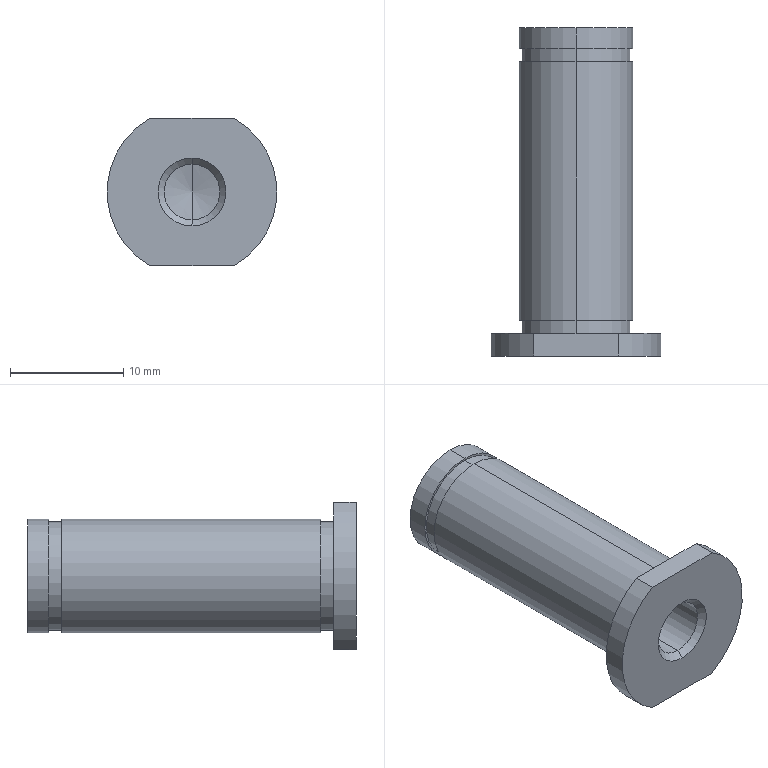Component | SolidWorks | MED02-10-Y2-F24.stp-1 | 1 solid | 24 faces | box 15 x 29 x 13 mm | volume 2240 mm3 | cylinder 12 | plane 8 | cone 4 | commonest cylinder face diameters 9.6 x4 10 x4 4.917 x2 15 x2 | material 45
STEP:
#1=COLOUR_RGB('',0.7922,0.8196,0.9333);
#2=FILL_AREA_STYLE_COLOUR('',#1);
#3=FILL_AREA_STYLE('',(#2));
#4=SURFACE_STYLE_FILL_AREA(#3);
#5=SURFACE_SIDE_STYLE('',(#4));
#6=SURFACE_STYLE_USAGE(.BOTH.,#5);
#7=PRESENTATION_STYLE_ASSIGNMENT((#6));
#8=CARTESIAN_POINT('',(0.5001,-0.1089,18.325));
#9=VERTEX_POINT('',#8);
#10=CARTESIAN_POINT('',(0.5001,-0.1089,18.703));
#11=VERTEX_POINT('',#10);
#12=CARTESIAN_POINT('',(0.5001,-0.1089,18.514));
#13=DIRECTION('',(0.,1.,0.));
#14=DIRECTION('',(0.,-0.,1.));
#15=AXIS2_PLACEMENT_3D('',#12,#13,#14);
#16=CIRCLE('',#15,0.189);
#17=EDGE_CURVE('',#9,#11,#16,.T.);
#18=ORIENTED_EDGE('',*,*,#17,.F.);
#19=CARTESIAN_POINT('',(0.5001,-0.1542,18.325));
#20=VERTEX_POINT('',#19);
#21=CARTESIAN_POINT('',(0.5001,-0.03607,18.325));
#22=DIRECTION('',(-0.,-1.,-0.));
#23=VECTOR('',#22,39.37);
#24=LINE('',#21,#23);
#25=EDGE_CURVE('',#9,#20,#24,.T.);
#26=ORIENTED_EDGE('',*,*,#25,.T.);
#27=CARTESIAN_POINT('',(0.5001,-0.1542,18.703));
#28=VERTEX_POINT('',#27);
#29=CARTESIAN_POINT('',(0.5001,-0.1542,18.514));
#30=DIRECTION('',(0.,1.,0.));
#31=DIRECTION('',(0.,-0.,1.));
#32=AXIS2_PLACEMENT_3D('',#29,#30,#31);
#33=CIRCLE('',#32,0.189);
#34=EDGE_CURVE('',#20,#28,#33,.T.);
#35=ORIENTED_EDGE('',*,*,#34,.T.);
#36=CARTESIAN_POINT('',(0.5001,-0.03607,18.703));
#37=DIRECTION('',(-0.,-1.,-0.));
#38=VECTOR('',#37,39.37);
#39=LINE('',#36,#38);
#40=EDGE_CURVE('',#11,#28,#39,.T.);
#41=ORIENTED_EDGE('',*,*,#40,.F.);
#42=EDGE_LOOP('',(#18,#26,#35,#41));
#43=FACE_OUTER_BOUND('',#42,.T.);
#44=CARTESIAN_POINT('',(0.5001,-0.03607,18.514));
#45=DIRECTION('',(-0.,-1.,-0.));
#46=DIRECTION('',(0.,-0.,1.));
#47=AXIS2_PLACEMENT_3D('',#44,#45,#46);
#48=CYLINDRICAL_SURFACE('',#47,0.189);
#49=ADVANCED_FACE('',(#43),#48,.T.);
#50=CARTESIAN_POINT('',(0.5001,-0.1542,18.317));
#51=VERTEX_POINT('',#50);
#52=CARTESIAN_POINT('',(0.5001,-0.1542,18.711));
#53=VERTEX_POINT('',#52);
#54=CARTESIAN_POINT('',(0.5001,-0.1542,18.514));
#55=DIRECTION('',(0.,1.,0.));
#56=DIRECTION('',(0.,-0.,1.));
#57=AXIS2_PLACEMENT_3D('',#54,#55,#56);
#58=CIRCLE('',#57,0.1969);
#59=EDGE_CURVE('',#51,#53,#58,.T.);
#60=ORIENTED_EDGE('',*,*,#59,.F.);
#61=CARTESIAN_POINT('',(0.5001,-1.054,18.317));
#62=VERTEX_POINT('',#61);
#63=CARTESIAN_POINT('',(0.5001,-0.03607,18.317));
#64=DIRECTION('',(-0.,-1.,-0.));
#65=VECTOR('',#64,39.37);
#66=LINE('',#63,#65);
#67=EDGE_CURVE('',#51,#62,#66,.T.);
#68=ORIENTED_EDGE('',*,*,#67,.T.);
#69=CARTESIAN_POINT('',(0.5001,-1.054,18.711));
#70=VERTEX_POINT('',#69);
#71=CARTESIAN_POINT('',(0.5001,-1.054,18.514));
#72=DIRECTION('',(0.,1.,0.));
#73=DIRECTION('',(0.,-0.,1.));
#74=AXIS2_PLACEMENT_3D('',#71,#72,#73);
#75=CIRCLE('',#74,0.1969);
#76=EDGE_CURVE('',#62,#70,#75,.T.);
#77=ORIENTED_EDGE('',*,*,#76,.T.);
#78=CARTESIAN_POINT('',(0.5001,-0.03607,18.711));
#79=DIRECTION('',(-0.,-1.,-0.));
#80=VECTOR('',#79,39.37);
#81=LINE('',#78,#80);
#82=EDGE_CURVE('',#53,#70,#81,.T.);
#83=ORIENTED_EDGE('',*,*,#82,.F.);
#84=EDGE_LOOP('',(#60,#68,#77,#83));
#85=FACE_OUTER_BOUND('',#84,.T.);
#86=CARTESIAN_POINT('',(0.5001,-0.03607,18.514));
#87=DIRECTION('',(-0.,-1.,-0.));
#88=DIRECTION('',(0.,-0.,1.));
#89=AXIS2_PLACEMENT_3D('',#86,#87,#88);
#90=CYLINDRICAL_SURFACE('',#89,0.1969);
#91=ADVANCED_FACE('',(#85),#90,.T.);
#92=CARTESIAN_POINT('',(0.5001,-1.156,18.417));
#93=VERTEX_POINT('',#92);
#94=CARTESIAN_POINT('',(0.5001,-1.156,18.61));
#95=VERTEX_POINT('',#94);
#96=CARTESIAN_POINT('',(0.5001,-1.156,18.514));
#97=DIRECTION('',(0.,1.,0.));
#98=DIRECTION('',(0.,0.,1.));
#99=AXIS2_PLACEMENT_3D('',#96,#97,#98);
#100=CIRCLE('',#99,0.09679);
#101=EDGE_CURVE('',#93,#95,#100,.T.);
#102=ORIENTED_EDGE('',*,*,#101,.T.);
#103=CARTESIAN_POINT('',(0.5001,-1.178,18.632));
#104=VERTEX_POINT('',#103);
#105=CARTESIAN_POINT('',(0.5001,-1.156,18.61));
#106=DIRECTION('',(0.,-0.7071,0.7071));
#107=VECTOR('',#106,39.37);
#108=LINE('',#105,#107);
#109=EDGE_CURVE('',#95,#104,#108,.T.);
#110=ORIENTED_EDGE('',*,*,#109,.T.);
#111=CARTESIAN_POINT('',(0.5001,-1.178,18.396));
#112=VERTEX_POINT('',#111);
#113=CARTESIAN_POINT('',(0.5001,-1.178,18.514));
#114=DIRECTION('',(0.,1.,0.));
#115=DIRECTION('',(0.,0.,1.));
#116=AXIS2_PLACEMENT_3D('',#113,#114,#115);
#117=CIRCLE('',#116,0.1181);
#118=EDGE_CURVE('',#112,#104,#117,.T.);
#119=ORIENTED_EDGE('',*,*,#118,.F.);
#120=CARTESIAN_POINT('',(0.5001,-1.156,18.417));
#121=DIRECTION('',(-0.,-0.7071,-0.7071));
#122=VECTOR('',#121,39.37);
#123=LINE('',#120,#122);
#124=EDGE_CURVE('',#93,#112,#123,.T.);
#125=ORIENTED_EDGE('',*,*,#124,.F.);
#126=EDGE_LOOP('',(#102,#110,#119,#125));
#127=FACE_OUTER_BOUND('',#126,.T.);
#128=CARTESIAN_POINT('',(0.5001,-1.156,18.514));
#129=DIRECTION('',(-0.,-1.,-0.));
#130=DIRECTION('',(-0.,0.,-1.));
#131=AXIS2_PLACEMENT_3D('',#128,#129,#130);
#132=CONICAL_SURFACE('',#131,0.09679,0.7854);
#133=ADVANCED_FACE('',(#127),#132,.F.);
#134=CARTESIAN_POINT('',(0.5001,-1.054,18.325));
#135=VERTEX_POINT('',#134);
#136=CARTESIAN_POINT('',(0.5001,-1.054,18.703));
#137=VERTEX_POINT('',#136);
#138=CARTESIAN_POINT('',(0.5001,-1.054,18.514));
#139=DIRECTION('',(0.,1.,0.));
#140=DIRECTION('',(0.,-0.,1.));
#141=AXIS2_PLACEMENT_3D('',#138,#139,#140);
#142=CIRCLE('',#141,0.189);
#143=EDGE_CURVE('',#135,#137,#142,.T.);
#144=ORIENTED_EDGE('',*,*,#143,.F.);
#145=CARTESIAN_POINT('',(0.5001,-1.099,18.325));
#146=VERTEX_POINT('',#145);
#147=CARTESIAN_POINT('',(0.5001,-0.03607,18.325));
#148=DIRECTION('',(-0.,-1.,-0.));
#149=VECTOR('',#148,39.37);
#150=LINE('',#147,#149);
#151=EDGE_CURVE('',#135,#146,#150,.T.);
#152=ORIENTED_EDGE('',*,*,#151,.T.);
#153=CARTESIAN_POINT('',(0.5001,-1.099,18.703));
#154=VERTEX_POINT('',#153);
#155=CARTESIAN_POINT('',(0.5001,-1.099,18.514));
#156=DIRECTION('',(0.,1.,0.));
#157=DIRECTION('',(0.,-0.,1.));
#158=AXIS2_PLACEMENT_3D('',#155,#156,#157);
#159=CIRCLE('',#158,0.189);
#160=EDGE_CURVE('',#146,#154,#159,.T.);
#161=ORIENTED_EDGE('',*,*,#160,.T.);
#162=CARTESIAN_POINT('',(0.5001,-0.03607,18.703));
#163=DIRECTION('',(-0.,-1.,-0.));
#164=VECTOR('',#163,39.37);
#165=LINE('',#162,#164);
#166=EDGE_CURVE('',#137,#154,#165,.T.);
#167=ORIENTED_EDGE('',*,*,#166,.F.);
#168=EDGE_LOOP('',(#144,#152,#161,#167));
#169=FACE_OUTER_BOUND('',#168,.T.);
#170=CARTESIAN_POINT('',(0.5001,-0.03607,18.514));
#171=DIRECTION('',(-0.,-1.,-0.));
#172=DIRECTION('',(0.,-0.,1.));
#173=AXIS2_PLACEMENT_3D('',#170,#171,#172);
#174=CYLINDRICAL_SURFACE('',#173,0.189);
#175=ADVANCED_FACE('',(#169),#174,.T.);
#176=CARTESIAN_POINT('',(0.5001,-0.7762,18.61));
#177=VERTEX_POINT('',#176);
#178=CARTESIAN_POINT('',(0.5001,-0.7762,18.417));
#179=VERTEX_POINT('',#178);
#180=CARTESIAN_POINT('',(0.5001,-0.7762,18.514));
#181=DIRECTION('',(0.,1.,0.));
#182=DIRECTION('',(0.,0.,1.));
#183=AXIS2_PLACEMENT_3D('',#180,#181,#182);
#184=CIRCLE('',#183,0.09679);
#185=EDGE_CURVE('',#177,#179,#184,.T.);
#186=ORIENTED_EDGE('',*,*,#185,.T.);
#187=CARTESIAN_POINT('',(0.5001,-0.03607,18.417));
#188=DIRECTION('',(-0.,-1.,-0.));
#189=VECTOR('',#188,39.37);
#190=LINE('',#187,#189);
#191=EDGE_CURVE('',#179,#93,#190,.T.);
#192=ORIENTED_EDGE('',*,*,#191,.T.);
#193=CARTESIAN_POINT('',(0.5001,-1.156,18.514));
#194=DIRECTION('',(0.,1.,0.));
#195=DIRECTION('',(0.,0.,1.));
#196=AXIS2_PLACEMENT_3D('',#193,#194,#195);
#197=CIRCLE('',#196,0.09679);
#198=EDGE_CURVE('',#95,#93,#197,.T.);
#199=ORIENTED_EDGE('',*,*,#198,.F.);
#200=CARTESIAN_POINT('',(0.5001,-0.03607,18.61));
#201=DIRECTION('',(-0.,-1.,-0.));
#202=VECTOR('',#201,39.37);
#203=LINE('',#200,#202);
#204=EDGE_CURVE('',#177,#95,#203,.T.);
#205=ORIENTED_EDGE('',*,*,#204,.F.);
#206=EDGE_LOOP('',(#186,#192,#199,#205));
#207=FACE_OUTER_BOUND('',#206,.T.);
#208=CARTESIAN_POINT('',(0.5001,-0.03607,18.514));
#209=DIRECTION('',(-0.,-1.,-0.));
#210=DIRECTION('',(0.,-0.,1.));
#211=AXIS2_PLACEMENT_3D('',#208,#209,#210);
#212=CYLINDRICAL_SURFACE('',#211,0.09679);
#213=ADVANCED_FACE('',(#207),#212,.F.);
#214=CARTESIAN_POINT('',(0.5001,-0.03607,18.317));
#215=VERTEX_POINT('',#214);
#216=CARTESIAN_POINT('',(0.5001,-0.03607,18.711));
#217=VERTEX_POINT('',#216);
#218=CARTESIAN_POINT('',(0.5001,-0.03607,18.514));
#219=DIRECTION('',(0.,1.,0.));
#220=DIRECTION('',(0.,-0.,1.));
#221=AXIS2_PLACEMENT_3D('',#218,#219,#220);
#222=CIRCLE('',#221,0.1969);
#223=EDGE_CURVE('',#215,#217,#222,.T.);
#224=ORIENTED_EDGE('',*,*,#223,.F.);
#225=CARTESIAN_POINT('',(0.5001,-0.1089,18.317));
#226=VERTEX_POINT('',#225);
#227=CARTESIAN_POINT('',(0.5001,-0.03607,18.317));
#228=DIRECTION('',(-0.,-1.,-0.));
#229=VECTOR('',#228,39.37);
#230=LINE('',#227,#229);
#231=EDGE_CURVE('',#215,#226,#230,.T.);
#232=ORIENTED_EDGE('',*,*,#231,.T.);
#233=CARTESIAN_POINT('',(0.5001,-0.1089,18.711));
#234=VERTEX_POINT('',#233);
#235=CARTESIAN_POINT('',(0.5001,-0.1089,18.514));
#236=DIRECTION('',(0.,1.,0.));
#237=DIRECTION('',(0.,-0.,1.));
#238=AXIS2_PLACEMENT_3D('',#235,#236,#237);
#239=CIRCLE('',#238,0.1969);
#240=EDGE_CURVE('',#226,#234,#239,.T.);
#241=ORIENTED_EDGE('',*,*,#240,.T.);
#242=CARTESIAN_POINT('',(0.5001,-0.03607,18.711));
#243=DIRECTION('',(-0.,-1.,-0.));
#244=VECTOR('',#243,39.37);
#245=LINE('',#242,#244);
#246=EDGE_CURVE('',#217,#234,#245,.T.);
#247=ORIENTED_EDGE('',*,*,#246,.F.);
#248=EDGE_LOOP('',(#224,#232,#241,#247));
#249=FACE_OUTER_BOUND('',#248,.T.);
#250=CARTESIAN_POINT('',(0.5001,-0.03607,18.514));
#251=DIRECTION('',(-0.,-1.,-0.));
#252=DIRECTION('',(0.,-0.,1.));
#253=AXIS2_PLACEMENT_3D('',#250,#251,#252);
#254=CYLINDRICAL_SURFACE('',#253,0.1969);
#255=ADVANCED_FACE('',(#249),#254,.T.);
#256=CARTESIAN_POINT('',(0.5001,-0.7565,18.514));
#257=VERTEX_POINT('',#256);
#258=CARTESIAN_POINT('',(0.5001,-8.603,-20.067));
#259=DIRECTION('',(-0.,-0.1993,-0.9799));
#260=VECTOR('',#259,39.37);
#261=LINE('',#258,#260);
#262=EDGE_CURVE('',#257,#179,#261,.T.);
#263=ORIENTED_EDGE('',*,*,#262,.F.);
#264=CARTESIAN_POINT('',(0.5001,-8.603,57.094));
#265=DIRECTION('',(0.,-0.1993,0.9799));
#266=VECTOR('',#265,39.37);
#267=LINE('',#264,#266);
#268=EDGE_CURVE('',#257,#177,#267,.T.);
#269=ORIENTED_EDGE('',*,*,#268,.T.);
#270=CARTESIAN_POINT('',(0.5001,-0.7762,18.514));
#271=DIRECTION('',(0.,1.,0.));
#272=DIRECTION('',(0.,0.,1.));
#273=AXIS2_PLACEMENT_3D('',#270,#271,#272);
#274=CIRCLE('',#273,0.09679);
#275=EDGE_CURVE('',#179,#177,#274,.T.);
#276=ORIENTED_EDGE('',*,*,#275,.F.);
#277=EDGE_LOOP('',(#263,#269,#276));
#278=FACE_OUTER_BOUND('',#277,.T.);
#279=CARTESIAN_POINT('',(0.5001,-8.603,18.514));
#280=DIRECTION('',(-0.,-1.,-0.));
#281=DIRECTION('',(-0.,0.,-1.));
#282=AXIS2_PLACEMENT_3D('',#279,#280,#281);
#283=CONICAL_SURFACE('',#282,38.58,1.37);
#284=ADVANCED_FACE('',(#278),#283,.F.);
#285=CARTESIAN_POINT('',(0.3528,-1.178,18.258));
#286=VERTEX_POINT('',#285);
#287=CARTESIAN_POINT('',(0.3528,-1.178,18.77));
#288=VERTEX_POINT('',#287);
#289=CARTESIAN_POINT('',(0.5001,-1.178,18.514));
#290=DIRECTION('',(0.,1.,0.));
#291=DIRECTION('',(0.,-0.,1.));
#292=AXIS2_PLACEMENT_3D('',#289,#290,#291);
#293=CIRCLE('',#292,0.2953);
#294=EDGE_CURVE('',#286,#288,#293,.T.);
#295=ORIENTED_EDGE('',*,*,#294,.T.);
#296=CARTESIAN_POINT('',(0.3528,-1.099,18.77));
#297=VERTEX_POINT('',#296);
#298=CARTESIAN_POINT('',(0.3528,-0.03607,18.77));
#299=DIRECTION('',(0.,1.,0.));
#300=VECTOR('',#299,39.37);
#301=LINE('',#298,#300);
#302=EDGE_CURVE('',#288,#297,#301,.T.);
#303=ORIENTED_EDGE('',*,*,#302,.T.);
#304=CARTESIAN_POINT('',(0.3528,-1.099,18.258));
#305=VERTEX_POINT('',#304);
#306=CARTESIAN_POINT('',(0.5001,-1.099,18.514));
#307=DIRECTION('',(0.,1.,0.));
#308=DIRECTION('',(0.,-0.,1.));
#309=AXIS2_PLACEMENT_3D('',#306,#307,#308);
#310=CIRCLE('',#309,0.2953);
#311=EDGE_CURVE('',#305,#297,#310,.T.);
#312=ORIENTED_EDGE('',*,*,#311,.F.);
#313=CARTESIAN_POINT('',(0.3528,-0.03607,18.258));
#314=DIRECTION('',(-0.,-1.,-0.));
#315=VECTOR('',#314,39.37);
#316=LINE('',#313,#315);
#317=EDGE_CURVE('',#305,#286,#316,.T.);
#318=ORIENTED_EDGE('',*,*,#317,.T.);
#319=EDGE_LOOP('',(#295,#303,#312,#318));
#320=FACE_OUTER_BOUND('',#319,.T.);
#321=CARTESIAN_POINT('',(0.5001,-0.03607,18.514));
#322=DIRECTION('',(-0.,-1.,-0.));
#323=DIRECTION('',(0.,-0.,1.));
#324=AXIS2_PLACEMENT_3D('',#321,#322,#323);
#325=CYLINDRICAL_SURFACE('',#324,0.2953);
#326=ADVANCED_FACE('',(#320),#325,.T.);
#327=ORIENTED_EDGE('',*,*,#268,.F.);
#328=ORIENTED_EDGE('',*,*,#262,.T.);
#329=ORIENTED_EDGE('',*,*,#185,.F.);
#330=EDGE_LOOP('',(#327,#328,#329));
#331=FACE_OUTER_BOUND('',#330,.T.);
#332=CARTESIAN_POINT('',(0.5001,-8.603,18.514));
#333=DIRECTION('',(-0.,-1.,-0.));
#334=DIRECTION('',(-0.,0.,-1.));
#335=AXIS2_PLACEMENT_3D('',#332,#333,#334);
#336=CONICAL_SURFACE('',#335,38.58,1.37);
#337=ADVANCED_FACE('',(#331),#336,.F.);
#338=CARTESIAN_POINT('',(0.6474,-1.178,18.77));
#339=VERTEX_POINT('',#338);
#340=CARTESIAN_POINT('',(0.2049,-1.178,18.77));
#341=DIRECTION('',(1.,-0.,-0.));
#342=VECTOR('',#341,39.37);
#343=LINE('',#340,#342);
#344=EDGE_CURVE('',#288,#339,#343,.T.);
#345=ORIENTED_EDGE('',*,*,#344,.T.);
#346=CARTESIAN_POINT('',(0.6474,-1.099,18.77));
#347=VERTEX_POINT('',#346);
#348=CARTESIAN_POINT('',(0.6474,-0.03607,18.77));
#349=DIRECTION('',(-0.,-1.,-0.));
#350=VECTOR('',#349,39.37);
#351=LINE('',#348,#350);
#352=EDGE_CURVE('',#347,#339,#351,.T.);
#353=ORIENTED_EDGE('',*,*,#352,.F.);
#354=CARTESIAN_POINT('',(0.7954,-1.099,18.77));
#355=DIRECTION('',(1.,-0.,-0.));
#356=VECTOR('',#355,39.37);
#357=LINE('',#354,#356);
#358=EDGE_CURVE('',#297,#347,#357,.T.);
#359=ORIENTED_EDGE('',*,*,#358,.F.);
#360=ORIENTED_EDGE('',*,*,#302,.F.);
#361=EDGE_LOOP('',(#345,#353,#359,#360));
#362=FACE_OUTER_BOUND('',#361,.T.);
#363=CARTESIAN_POINT('',(0.2049,-1.099,18.77));
#364=DIRECTION('',(-0.,0.,-1.));
#365=DIRECTION('',(1.,-0.,-0.));
#366=AXIS2_PLACEMENT_3D('',#363,#364,#365);
#367=PLANE('',#366);
#368=ADVANCED_FACE('',(#362),#367,.F.);
#369=CARTESIAN_POINT('',(0.6474,-1.178,18.258));
#370=VERTEX_POINT('',#369);
#371=CARTESIAN_POINT('',(0.5001,-1.178,18.514));
#372=DIRECTION('',(0.,1.,0.));
#373=DIRECTION('',(0.,-0.,1.));
#374=AXIS2_PLACEMENT_3D('',#371,#372,#373);
#375=CIRCLE('',#374,0.2953);
#376=EDGE_CURVE('',#339,#370,#375,.T.);
#377=ORIENTED_EDGE('',*,*,#376,.F.);
#378=ORIENTED_EDGE('',*,*,#344,.F.);
#379=ORIENTED_EDGE('',*,*,#294,.F.);
#380=CARTESIAN_POINT('',(0.7954,-1.178,18.258));
#381=DIRECTION('',(-1.,0.,0.));
#382=VECTOR('',#381,39.37);
#383=LINE('',#380,#382);
#384=EDGE_CURVE('',#370,#286,#383,.T.);
#385=ORIENTED_EDGE('',*,*,#384,.F.);
#386=EDGE_LOOP('',(#377,#378,#379,#385));
#387=FACE_OUTER_BOUND('',#386,.T.);
#388=ORIENTED_EDGE('',*,*,#118,.T.);
#389=CARTESIAN_POINT('',(0.5001,-1.178,18.514));
#390=DIRECTION('',(0.,1.,0.));
#391=DIRECTION('',(0.,0.,1.));
#392=AXIS2_PLACEMENT_3D('',#389,#390,#391);
#393=CIRCLE('',#392,0.1181);
#394=EDGE_CURVE('',#104,#112,#393,.T.);
#395=ORIENTED_EDGE('',*,*,#394,.T.);
#396=EDGE_LOOP('',(#388,#395));
#397=FACE_BOUND('',#396,.T.);
#398=CARTESIAN_POINT('',(0.6182,-1.178,18.514));
#399=DIRECTION('',(0.,1.,0.));
#400=DIRECTION('',(-1.,0.,0.));
#401=AXIS2_PLACEMENT_3D('',#398,#399,#400);
#402=PLANE('',#401);
#403=ADVANCED_FACE('',(#387,#397),#402,.F.);
#404=ORIENTED_EDGE('',*,*,#311,.T.);
#405=ORIENTED_EDGE('',*,*,#358,.T.);
#406=CARTESIAN_POINT('',(0.6474,-1.099,18.258));
#407=VERTEX_POINT('',#406);
#408=CARTESIAN_POINT('',(0.5001,-1.099,18.514));
#409=DIRECTION('',(0.,1.,0.));
#410=DIRECTION('',(0.,-0.,1.));
#411=AXIS2_PLACEMENT_3D('',#408,#409,#410);
#412=CIRCLE('',#411,0.2953);
#413=EDGE_CURVE('',#347,#407,#412,.T.);
#414=ORIENTED_EDGE('',*,*,#413,.T.);
#415=CARTESIAN_POINT('',(0.7954,-1.099,18.258));
#416=DIRECTION('',(-1.,0.,0.));
#417=VECTOR('',#416,39.37);
#418=LINE('',#415,#417);
#419=EDGE_CURVE('',#407,#305,#418,.T.);
#420=ORIENTED_EDGE('',*,*,#419,.T.);
#421=EDGE_LOOP('',(#404,#405,#414,#420));
#422=FACE_OUTER_BOUND('',#421,.T.);
#423=CARTESIAN_POINT('',(0.5001,-1.099,18.514));
#424=DIRECTION('',(0.,1.,0.));
#425=DIRECTION('',(0.,-0.,1.));
#426=AXIS2_PLACEMENT_3D('',#423,#424,#425);
#427=CIRCLE('',#426,0.189);
#428=EDGE_CURVE('',#154,#146,#427,.T.);
#429=ORIENTED_EDGE('',*,*,#428,.F.);
#430=ORIENTED_EDGE('',*,*,#160,.F.);
#431=EDGE_LOOP('',(#429,#430));
#432=FACE_BOUND('',#431,.T.);
#433=CARTESIAN_POINT('',(0.7954,-1.099,18.514));
#434=DIRECTION('',(-0.,-1.,-0.));
#435=DIRECTION('',(-0.,0.,-1.));
#436=AXIS2_PLACEMENT_3D('',#433,#434,#435);
#437=PLANE('',#436);
#438=ADVANCED_FACE('',(#422,#432),#437,.F.);
#439=ORIENTED_EDGE('',*,*,#376,.T.);
#440=CARTESIAN_POINT('',(0.6474,-0.03607,18.258));
#441=DIRECTION('',(0.,1.,0.));
#442=VECTOR('',#441,39.37);
#443=LINE('',#440,#442);
#444=EDGE_CURVE('',#370,#407,#443,.T.);
#445=ORIENTED_EDGE('',*,*,#444,.T.);
#446=ORIENTED_EDGE('',*,*,#413,.F.);
#447=ORIENTED_EDGE('',*,*,#352,.T.);
#448=EDGE_LOOP('',(#439,#445,#446,#447));
#449=FACE_OUTER_BOUND('',#448,.T.);
#450=CARTESIAN_POINT('',(0.5001,-0.03607,18.514));
#451=DIRECTION('',(-0.,-1.,-0.));
#452=DIRECTION('',(0.,-0.,1.));
#453=AXIS2_PLACEMENT_3D('',#450,#451,#452);
#454=CYLINDRICAL_SURFACE('',#453,0.2953);
#455=ADVANCED_FACE('',(#449),#454,.T.);
#456=ORIENTED_EDGE('',*,*,#384,.T.);
#457=ORIENTED_EDGE('',*,*,#317,.F.);
#458=ORIENTED_EDGE('',*,*,#419,.F.);
#459=ORIENTED_EDGE('',*,*,#444,.F.);
#460=EDGE_LOOP('',(#456,#457,#458,#459));
#461=FACE_OUTER_BOUND('',#460,.T.);
#462=CARTESIAN_POINT('',(0.7954,-1.099,18.258));
#463=DIRECTION('',(0.,-0.,1.));
#464=DIRECTION('',(-0.,-1.,-0.));
#465=AXIS2_PLACEMENT_3D('',#462,#463,#464);
#466=PLANE('',#465);
#467=ADVANCED_FACE('',(#461),#466,.F.);
#468=CARTESIAN_POINT('',(0.5001,-0.03607,18.514));
#469=DIRECTION('',(0.,1.,0.));
#470=DIRECTION('',(0.,-0.,1.));
#471=AXIS2_PLACEMENT_3D('',#468,#469,#470);
#472=CIRCLE('',#471,0.1969);
#473=EDGE_CURVE('',#217,#215,#472,.T.);
#474=ORIENTED_EDGE('',*,*,#473,.T.);
#475=ORIENTED_EDGE('',*,*,#223,.T.);
#476=EDGE_LOOP('',(#474,#475));
#477=FACE_OUTER_BOUND('',#476,.T.);
#478=CARTESIAN_POINT('',(0.697,-0.03607,18.514));
#479=DIRECTION('',(-0.,-1.,-0.));
#480=DIRECTION('',(-0.,0.,-1.));
#481=AXIS2_PLACEMENT_3D('',#478,#479,#480);
#482=PLANE('',#481);
#483=ADVANCED_FACE('',(#477),#482,.F.);
#484=ORIENTED_EDGE('',*,*,#231,.F.);
#485=ORIENTED_EDGE('',*,*,#473,.F.);
#486=ORIENTED_EDGE('',*,*,#246,.T.);
#487=CARTESIAN_POINT('',(0.5001,-0.1089,18.514));
#488=DIRECTION('',(0.,1.,0.));
#489=DIRECTION('',(0.,-0.,1.));
#490=AXIS2_PLACEMENT_3D('',#487,#488,#489);
#491=CIRCLE('',#490,0.1969);
#492=EDGE_CURVE('',#234,#226,#491,.T.);
#493=ORIENTED_EDGE('',*,*,#492,.T.);
#494=EDGE_LOOP('',(#484,#485,#486,#493));
#495=FACE_OUTER_BOUND('',#494,.T.);
#496=CARTESIAN_POINT('',(0.5001,-0.03607,18.514));
#497=DIRECTION('',(-0.,-1.,-0.));
#498=DIRECTION('',(0.,-0.,1.));
#499=AXIS2_PLACEMENT_3D('',#496,#497,#498);
#500=CYLINDRICAL_SURFACE('',#499,0.1969);
#501=ADVANCED_FACE('',(#495),#500,.T.);
#502=ORIENTED_EDGE('',*,*,#191,.F.);
#503=ORIENTED_EDGE('',*,*,#275,.T.);
#504=ORIENTED_EDGE('',*,*,#204,.T.);
#505=ORIENTED_EDGE('',*,*,#101,.F.);
#506=EDGE_LOOP('',(#502,#503,#504,#505));
#507=FACE_OUTER_BOUND('',#506,.T.);
#508=CARTESIAN_POINT('',(0.5001,-0.03607,18.514));
#509=DIRECTION('',(-0.,-1.,-0.));
#510=DIRECTION('',(0.,-0.,1.));
#511=AXIS2_PLACEMENT_3D('',#508,#509,#510);
#512=CYLINDRICAL_SURFACE('',#511,0.09679);
#513=ADVANCED_FACE('',(#507),#512,.F.);
#514=ORIENTED_EDGE('',*,*,#151,.F.);
#515=CARTESIAN_POINT('',(0.5001,-1.054,18.514));
#516=DIRECTION('',(0.,1.,0.));
#517=DIRECTION('',(0.,-0.,1.));
#518=AXIS2_PLACEMENT_3D('',#515,#516,#517);
#519=CIRCLE('',#518,0.189);
#520=EDGE_CURVE('',#137,#135,#519,.T.);
#521=ORIENTED_EDGE('',*,*,#520,.F.);
#522=ORIENTED_EDGE('',*,*,#166,.T.);
#523=ORIENTED_EDGE('',*,*,#428,.T.);
#524=EDGE_LOOP('',(#514,#521,#522,#523));
#525=FACE_OUTER_BOUND('',#524,.T.);
#526=CARTESIAN_POINT('',(0.5001,-0.03607,18.514));
#527=DIRECTION('',(-0.,-1.,-0.));
#528=DIRECTION('',(0.,-0.,1.));
#529=AXIS2_PLACEMENT_3D('',#526,#527,#528);
#530=CYLINDRICAL_SURFACE('',#529,0.189);
#531=ADVANCED_FACE('',(#525),#530,.T.);
#532=ORIENTED_EDGE('',*,*,#109,.F.);
#533=ORIENTED_EDGE('',*,*,#198,.T.);
#534=ORIENTED_EDGE('',*,*,#124,.T.);
#535=ORIENTED_EDGE('',*,*,#394,.F.);
#536=EDGE_LOOP('',(#532,#533,#534,#535));
#537=FACE_OUTER_BOUND('',#536,.T.);
#538=CARTESIAN_POINT('',(0.5001,-1.156,18.514));
#539=DIRECTION('',(-0.,-1.,-0.));
#540=DIRECTION('',(-0.,0.,-1.));
#541=AXIS2_PLACEMENT_3D('',#538,#539,#540);
#542=CONICAL_SURFACE('',#541,0.09679,0.7854);
#543=ADVANCED_FACE('',(#537),#542,.F.);
#544=CARTESIAN_POINT('',(0.5001,-1.054,18.514));
#545=DIRECTION('',(0.,1.,0.));
#546=DIRECTION('',(0.,-0.,1.));
#547=AXIS2_PLACEMENT_3D('',#544,#545,#546);
#548=CIRCLE('',#547,0.1969);
#549=EDGE_CURVE('',#70,#62,#548,.T.);
#550=ORIENTED_EDGE('',*,*,#549,.F.);
#551=ORIENTED_EDGE('',*,*,#76,.F.);
#552=EDGE_LOOP('',(#550,#551));
#553=FACE_OUTER_BOUND('',#552,.T.);
#554=ORIENTED_EDGE('',*,*,#520,.T.);
#555=ORIENTED_EDGE('',*,*,#143,.T.);
#556=EDGE_LOOP('',(#554,#555));
#557=FACE_BOUND('',#556,.T.);
#558=CARTESIAN_POINT('',(0.6891,-1.054,18.514));
#559=DIRECTION('',(0.,1.,0.));
#560=DIRECTION('',(-1.,0.,0.));
#561=AXIS2_PLACEMENT_3D('',#558,#559,#560);
#562=PLANE('',#561);
#563=ADVANCED_FACE('',(#553,#557),#562,.F.);
#564=ORIENTED_EDGE('',*,*,#67,.F.);
#565=CARTESIAN_POINT('',(0.5001,-0.1542,18.514));
#566=DIRECTION('',(0.,1.,0.));
#567=DIRECTION('',(0.,-0.,1.));
#568=AXIS2_PLACEMENT_3D('',#565,#566,#567);
#569=CIRCLE('',#568,0.1969);
#570=EDGE_CURVE('',#53,#51,#569,.T.);
#571=ORIENTED_EDGE('',*,*,#570,.F.);
#572=ORIENTED_EDGE('',*,*,#82,.T.);
#573=ORIENTED_EDGE('',*,*,#549,.T.);
#574=EDGE_LOOP('',(#564,#571,#572,#573));
#575=FACE_OUTER_BOUND('',#574,.T.);
#576=CARTESIAN_POINT('',(0.5001,-0.03607,18.514));
#577=DIRECTION('',(-0.,-1.,-0.));
#578=DIRECTION('',(0.,-0.,1.));
#579=AXIS2_PLACEMENT_3D('',#576,#577,#578);
#580=CYLINDRICAL_SURFACE('',#579,0.1969);
#581=ADVANCED_FACE('',(#575),#580,.T.);
#582=ORIENTED_EDGE('',*,*,#570,.T.);
#583=ORIENTED_EDGE('',*,*,#59,.T.);
#584=EDGE_LOOP('',(#582,#583));
#585=FACE_OUTER_BOUND('',#584,.T.);
#586=CARTESIAN_POINT('',(0.5001,-0.1542,18.514));
#587=DIRECTION('',(0.,1.,0.));
#588=DIRECTION('',(0.,-0.,1.));
#589=AXIS2_PLACEMENT_3D('',#586,#587,#588);
#590=CIRCLE('',#589,0.189);
#591=EDGE_CURVE('',#28,#20,#590,.T.);
#592=ORIENTED_EDGE('',*,*,#591,.F.);
#593=ORIENTED_EDGE('',*,*,#34,.F.);
#594=EDGE_LOOP('',(#592,#593));
#595=FACE_BOUND('',#594,.T.);
#596=CARTESIAN_POINT('',(0.697,-0.1542,18.514));
#597=DIRECTION('',(-0.,-1.,-0.));
#598=DIRECTION('',(-0.,0.,-1.));
#599=AXIS2_PLACEMENT_3D('',#596,#597,#598);
#600=PLANE('',#599);
#601=ADVANCED_FACE('',(#585,#595),#600,.F.);
#602=ORIENTED_EDGE('',*,*,#25,.F.);
#603=CARTESIAN_POINT('',(0.5001,-0.1089,18.514));
#604=DIRECTION('',(0.,1.,0.));
#605=DIRECTION('',(0.,-0.,1.));
#606=AXIS2_PLACEMENT_3D('',#603,#604,#605);
#607=CIRCLE('',#606,0.189);
#608=EDGE_CURVE('',#11,#9,#607,.T.);
#609=ORIENTED_EDGE('',*,*,#608,.F.);
#610=ORIENTED_EDGE('',*,*,#40,.T.);
#611=ORIENTED_EDGE('',*,*,#591,.T.);
#612=EDGE_LOOP('',(#602,#609,#610,#611));
#613=FACE_OUTER_BOUND('',#612,.T.);
#614=CARTESIAN_POINT('',(0.5001,-0.03607,18.514));
#615=DIRECTION('',(-0.,-1.,-0.));
#616=DIRECTION('',(0.,-0.,1.));
#617=AXIS2_PLACEMENT_3D('',#614,#615,#616);
#618=CYLINDRICAL_SURFACE('',#617,0.189);
#619=ADVANCED_FACE('',(#613),#618,.T.);
#620=ORIENTED_EDGE('',*,*,#492,.F.);
#621=ORIENTED_EDGE('',*,*,#240,.F.);
#622=EDGE_LOOP('',(#620,#621));
#623=FACE_OUTER_BOUND('',#622,.T.);
#624=ORIENTED_EDGE('',*,*,#608,.T.);
#625=ORIENTED_EDGE('',*,*,#17,.T.);
#626=EDGE_LOOP('',(#624,#625));
#627=FACE_BOUND('',#626,.T.);
#628=CARTESIAN_POINT('',(0.6891,-0.1089,18.514));
#629=DIRECTION('',(0.,1.,0.));
#630=DIRECTION('',(-1.,0.,0.));
#631=AXIS2_PLACEMENT_3D('',#628,#629,#630);
#632=PLANE('',#631);
#633=ADVANCED_FACE('',(#623,#627),#632,.F.);
#634=CLOSED_SHELL('',(#49,#91,#133,#175,#213,#255,#284,#326,#337,#368,#403,#438,#455,#467,#483,#501,#513,#531,#543,#563,#581,#601,#619,#633));
#635=MANIFOLD_SOLID_BREP('',#634);
#636=STYLED_ITEM('',(#7),#635);
#637=PRESENTATION_LAYER_ASSIGNMENT('','',(#636));
#638=(LENGTH_UNIT()NAMED_UNIT(*)SI_UNIT($,.METRE.));
#639=LENGTH_MEASURE_WITH_UNIT(LENGTH_MEASURE(0.0254),#638);
#640=DIMENSIONAL_EXPONENTS(1.,0.,0.,0.,0.,0.,0.);
#641=(CONVERSION_BASED_UNIT('',#639)LENGTH_UNIT()NAMED_UNIT(#640));
#642=UNCERTAINTY_MEASURE_WITH_UNIT(LENGTH_MEASURE(0.00001),#641,'','');
#643=(NAMED_UNIT(*)PLANE_ANGLE_UNIT()SI_UNIT($,.RADIAN.));
#644=(NAMED_UNIT(*)SI_UNIT($,.STERADIAN.)SOLID_ANGLE_UNIT());
#645=(GEOMETRIC_REPRESENTATION_CONTEXT(3)GLOBAL_UNCERTAINTY_ASSIGNED_CONTEXT((#642))GLOBAL_UNIT_ASSIGNED_CONTEXT((#641,#643,#644))REPRESENTATION_CONTEXT('',''));
#646=MECHANICAL_DESIGN_GEOMETRIC_PRESENTATION_REPRESENTATION('',(#636),#645);
#647=CARTESIAN_POINT('',(0.,0.,0.));
#648=DIRECTION('',(0.,0.,1.));
#649=DIRECTION('',(1.,0.,0.));
#650=AXIS2_PLACEMENT_3D('',#647,#648,#649);
#651=(LENGTH_UNIT()NAMED_UNIT(*)SI_UNIT($,.METRE.));
#652=LENGTH_MEASURE_WITH_UNIT(LENGTH_MEASURE(0.0254),#651);
#653=DIMENSIONAL_EXPONENTS(1.,0.,0.,0.,0.,0.,0.);
#654=(CONVERSION_BASED_UNIT('',#652)LENGTH_UNIT()NAMED_UNIT(#653));
#655=UNCERTAINTY_MEASURE_WITH_UNIT(LENGTH_MEASURE(0.00001),#654,'','');
#656=(NAMED_UNIT(*)PLANE_ANGLE_UNIT()SI_UNIT($,.RADIAN.));
#657=(NAMED_UNIT(*)SI_UNIT($,.STERADIAN.)SOLID_ANGLE_UNIT());
#658=(GEOMETRIC_REPRESENTATION_CONTEXT(3)GLOBAL_UNCERTAINTY_ASSIGNED_CONTEXT((#655))GLOBAL_UNIT_ASSIGNED_CONTEXT((#654,#656,#657))REPRESENTATION_CONTEXT('',''));
#659=ADVANCED_BREP_SHAPE_REPRESENTATION('',(#635,#650),#658);